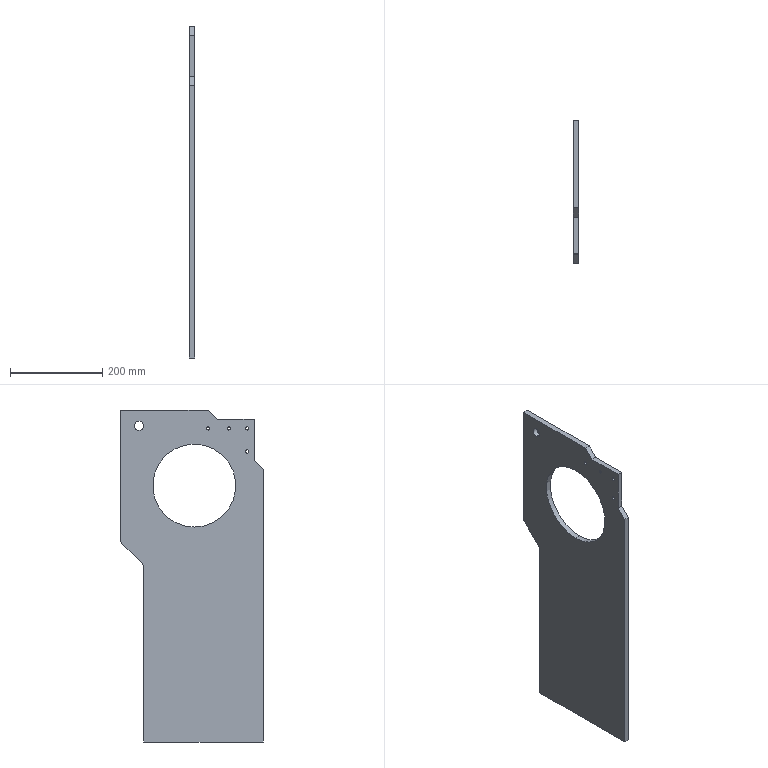Component | SolidWorks | JHK-A1003DriveWheelSupportPlateRight-3 | 1 solid | 28 faces | box 12 x 310 x 720 mm | volume 2071677 mm3 | cylinder 14 | plane 12 | cone 2 | commonest cylinder face diameters 6.8 x8 20 x4 180 x2 | material Q235A
build123d program:
from build123d import *

# Parameters (mm, degrees)
BOSS_EXTRUDE1_DEPTH = 6
SKETCH2_R           = 90
SKETCH2_R_2         = 10
CUT_EXTRUDE1_DEPTH  = 397.729
M8_TAPPED_HOLE1_D   = 6.8
FILLET1_R           = 10
CHAMFER1_SIZE       = 1.2


with BuildPart() as part:
    # Sketch1 → Boss-Extrude1 (new, symmetric)
    with BuildSketch(Plane(origin=(0, 0, 0), x_dir=(0, 0, -1), z_dir=(1, 0, 0))):
        Polygon((-355, 155), (-69, 155), (-19, 105), (365, 105), (365, -155), (-225, -155), (-245, -135), (-335, -135), (-335, -55), (-355, -35), align=None)
    extrude(amount=BOSS_EXTRUDE1_DEPTH, both=True)

    # Sketch2 → Cut-Extrude1 (cut, through all)
    with BuildSketch(Plane(origin=(6, 0, 0), x_dir=(0, 0, -1), z_dir=(1, 0, 0))):
        with Locations((-191, -5)):
            Circle(SKETCH2_R)
        with Locations((-321, 115)):
            Circle(SKETCH2_R_2)
    extrude(amount=-CUT_EXTRUDE1_DEPTH, mode=Mode.SUBTRACT)

    # M8 Tapped Hole1 (through all)
    with Locations(Plane(origin=(6, 0, 0), x_dir=(0, 0, -1), z_dir=(1, 0, 0))):
        with Locations((-315, -120), (-265, -120), (-315, -80), (-315, -35)):
            Hole(M8_TAPPED_HOLE1_D / 2)

    # Fillet1
    fillet1_edges = [part.edges().sort_by_distance(p)[0] for p in [
        (0, 155, 69),
        (0, 105, 19),
    ]]
    fillet(fillet1_edges, radius=FILLET1_R)

    # Chamfer1
    chamfer1_edges = [part.edges().sort_by_distance(p)[0] for p in [
        (6, 115, 331),
    ]]
    chamfer(chamfer1_edges, length=CHAMFER1_SIZE)


solid = part.part

# Placed as in the assembly
solid = solid.moved(Location((79, 0, 0), (0, 0, 0)))
STEP:
#1=CARTESIAN_POINT('',(3.299,4.528,13.031));
#2=VERTEX_POINT('',#1);
#3=CARTESIAN_POINT('',(3.299,4.528,12.244));
#4=VERTEX_POINT('',#3);
#5=CARTESIAN_POINT('',(3.299,4.528,12.638));
#6=DIRECTION('',(1.,0.,0.));
#7=DIRECTION('',(0.,0.,1.));
#8=AXIS2_PLACEMENT_3D('',#5,#6,#7);
#9=CIRCLE('',#8,0.3937);
#10=EDGE_CURVE('',#2,#4,#9,.T.);
#11=ORIENTED_EDGE('',*,*,#10,.F.);
#12=CARTESIAN_POINT('',(3.346,4.528,13.079));
#13=VERTEX_POINT('',#12);
#14=CARTESIAN_POINT('',(3.299,4.528,13.031));
#15=DIRECTION('',(0.7071,0.,0.7071));
#16=VECTOR('',#15,39.37);
#17=LINE('',#14,#16);
#18=EDGE_CURVE('',#2,#13,#17,.T.);
#19=ORIENTED_EDGE('',*,*,#18,.T.);
#20=CARTESIAN_POINT('',(3.346,4.528,12.197));
#21=VERTEX_POINT('',#20);
#22=CARTESIAN_POINT('',(3.346,4.528,12.638));
#23=DIRECTION('',(-1.,0.,0.));
#24=DIRECTION('',(0.,0.,1.));
#25=AXIS2_PLACEMENT_3D('',#22,#23,#24);
#26=CIRCLE('',#25,0.4409);
#27=EDGE_CURVE('',#21,#13,#26,.T.);
#28=ORIENTED_EDGE('',*,*,#27,.F.);
#29=CARTESIAN_POINT('',(3.299,4.528,12.244));
#30=DIRECTION('',(0.7071,0.,-0.7071));
#31=VECTOR('',#30,39.37);
#32=LINE('',#29,#31);
#33=EDGE_CURVE('',#4,#21,#32,.T.);
#34=ORIENTED_EDGE('',*,*,#33,.F.);
#35=EDGE_LOOP('',(#11,#19,#28,#34));
#36=FACE_OUTER_BOUND('',#35,.T.);
#37=CARTESIAN_POINT('',(3.299,4.528,12.638));
#38=DIRECTION('',(1.,0.,0.));
#39=DIRECTION('',(0.,0.,-1.));
#40=AXIS2_PLACEMENT_3D('',#37,#38,#39);
#41=CONICAL_SURFACE('',#40,0.3937,0.7854);
#42=ADVANCED_FACE('',(#36),#41,.F.);
#43=CARTESIAN_POINT('',(2.874,-4.724,12.535));
#44=VERTEX_POINT('',#43);
#45=CARTESIAN_POINT('',(2.874,-4.724,12.268));
#46=VERTEX_POINT('',#45);
#47=CARTESIAN_POINT('',(2.874,-4.724,12.402));
#48=DIRECTION('',(1.,0.,0.));
#49=DIRECTION('',(0.,0.,-1.));
#50=AXIS2_PLACEMENT_3D('',#47,#48,#49);
#51=CIRCLE('',#50,0.1339);
#52=EDGE_CURVE('',#44,#46,#51,.T.);
#53=ORIENTED_EDGE('',*,*,#52,.F.);
#54=CARTESIAN_POINT('',(3.346,-4.724,12.535));
#55=VERTEX_POINT('',#54);
#56=CARTESIAN_POINT('',(3.346,-4.724,12.535));
#57=DIRECTION('',(1.,0.,0.));
#58=VECTOR('',#57,39.37);
#59=LINE('',#56,#58);
#60=EDGE_CURVE('',#44,#55,#59,.T.);
#61=ORIENTED_EDGE('',*,*,#60,.T.);
#62=CARTESIAN_POINT('',(3.346,-4.724,12.268));
#63=VERTEX_POINT('',#62);
#64=CARTESIAN_POINT('',(3.346,-4.724,12.402));
#65=DIRECTION('',(1.,0.,0.));
#66=DIRECTION('',(0.,0.,-1.));
#67=AXIS2_PLACEMENT_3D('',#64,#65,#66);
#68=CIRCLE('',#67,0.1339);
#69=EDGE_CURVE('',#55,#63,#68,.T.);
#70=ORIENTED_EDGE('',*,*,#69,.T.);
#71=CARTESIAN_POINT('',(3.346,-4.724,12.268));
#72=DIRECTION('',(1.,0.,0.));
#73=VECTOR('',#72,39.37);
#74=LINE('',#71,#73);
#75=EDGE_CURVE('',#46,#63,#74,.T.);
#76=ORIENTED_EDGE('',*,*,#75,.F.);
#77=EDGE_LOOP('',(#53,#61,#70,#76));
#78=FACE_OUTER_BOUND('',#77,.T.);
#79=CARTESIAN_POINT('',(3.346,-4.724,12.402));
#80=DIRECTION('',(1.,0.,0.));
#81=DIRECTION('',(0.,0.,-1.));
#82=AXIS2_PLACEMENT_3D('',#79,#80,#81);
#83=CYLINDRICAL_SURFACE('',#82,0.1339);
#84=ADVANCED_FACE('',(#78),#83,.F.);
#85=CARTESIAN_POINT('',(2.874,-4.724,10.567));
#86=VERTEX_POINT('',#85);
#87=CARTESIAN_POINT('',(2.874,-4.724,10.299));
#88=VERTEX_POINT('',#87);
#89=CARTESIAN_POINT('',(2.874,-4.724,10.433));
#90=DIRECTION('',(1.,0.,0.));
#91=DIRECTION('',(0.,0.,-1.));
#92=AXIS2_PLACEMENT_3D('',#89,#90,#91);
#93=CIRCLE('',#92,0.1339);
#94=EDGE_CURVE('',#86,#88,#93,.T.);
#95=ORIENTED_EDGE('',*,*,#94,.F.);
#96=CARTESIAN_POINT('',(3.346,-4.724,10.567));
#97=VERTEX_POINT('',#96);
#98=CARTESIAN_POINT('',(3.346,-4.724,10.567));
#99=DIRECTION('',(1.,0.,0.));
#100=VECTOR('',#99,39.37);
#101=LINE('',#98,#100);
#102=EDGE_CURVE('',#86,#97,#101,.T.);
#103=ORIENTED_EDGE('',*,*,#102,.T.);
#104=CARTESIAN_POINT('',(3.346,-4.724,10.299));
#105=VERTEX_POINT('',#104);
#106=CARTESIAN_POINT('',(3.346,-4.724,10.433));
#107=DIRECTION('',(1.,0.,0.));
#108=DIRECTION('',(0.,0.,-1.));
#109=AXIS2_PLACEMENT_3D('',#106,#107,#108);
#110=CIRCLE('',#109,0.1339);
#111=EDGE_CURVE('',#97,#105,#110,.T.);
#112=ORIENTED_EDGE('',*,*,#111,.T.);
#113=CARTESIAN_POINT('',(3.346,-4.724,10.299));
#114=DIRECTION('',(1.,0.,0.));
#115=VECTOR('',#114,39.37);
#116=LINE('',#113,#115);
#117=EDGE_CURVE('',#88,#105,#116,.T.);
#118=ORIENTED_EDGE('',*,*,#117,.F.);
#119=EDGE_LOOP('',(#95,#103,#112,#118));
#120=FACE_OUTER_BOUND('',#119,.T.);
#121=CARTESIAN_POINT('',(3.346,-4.724,10.433));
#122=DIRECTION('',(1.,0.,0.));
#123=DIRECTION('',(0.,0.,-1.));
#124=AXIS2_PLACEMENT_3D('',#121,#122,#123);
#125=CYLINDRICAL_SURFACE('',#124,0.1339);
#126=ADVANCED_FACE('',(#120),#125,.F.);
#127=CARTESIAN_POINT('',(2.874,-3.15,12.535));
#128=VERTEX_POINT('',#127);
#129=CARTESIAN_POINT('',(2.874,-3.15,12.268));
#130=VERTEX_POINT('',#129);
#131=CARTESIAN_POINT('',(2.874,-3.15,12.402));
#132=DIRECTION('',(1.,0.,0.));
#133=DIRECTION('',(0.,0.,-1.));
#134=AXIS2_PLACEMENT_3D('',#131,#132,#133);
#135=CIRCLE('',#134,0.1339);
#136=EDGE_CURVE('',#128,#130,#135,.T.);
#137=ORIENTED_EDGE('',*,*,#136,.F.);
#138=CARTESIAN_POINT('',(3.346,-3.15,12.535));
#139=VERTEX_POINT('',#138);
#140=CARTESIAN_POINT('',(3.346,-3.15,12.535));
#141=DIRECTION('',(1.,0.,0.));
#142=VECTOR('',#141,39.37);
#143=LINE('',#140,#142);
#144=EDGE_CURVE('',#128,#139,#143,.T.);
#145=ORIENTED_EDGE('',*,*,#144,.T.);
#146=CARTESIAN_POINT('',(3.346,-3.15,12.268));
#147=VERTEX_POINT('',#146);
#148=CARTESIAN_POINT('',(3.346,-3.15,12.402));
#149=DIRECTION('',(1.,0.,0.));
#150=DIRECTION('',(0.,0.,-1.));
#151=AXIS2_PLACEMENT_3D('',#148,#149,#150);
#152=CIRCLE('',#151,0.1339);
#153=EDGE_CURVE('',#139,#147,#152,.T.);
#154=ORIENTED_EDGE('',*,*,#153,.T.);
#155=CARTESIAN_POINT('',(3.346,-3.15,12.268));
#156=DIRECTION('',(1.,0.,0.));
#157=VECTOR('',#156,39.37);
#158=LINE('',#155,#157);
#159=EDGE_CURVE('',#130,#147,#158,.T.);
#160=ORIENTED_EDGE('',*,*,#159,.F.);
#161=EDGE_LOOP('',(#137,#145,#154,#160));
#162=FACE_OUTER_BOUND('',#161,.T.);
#163=CARTESIAN_POINT('',(3.346,-3.15,12.402));
#164=DIRECTION('',(1.,0.,0.));
#165=DIRECTION('',(0.,0.,-1.));
#166=AXIS2_PLACEMENT_3D('',#163,#164,#165);
#167=CYLINDRICAL_SURFACE('',#166,0.1339);
#168=ADVANCED_FACE('',(#162),#167,.F.);
#169=CARTESIAN_POINT('',(2.874,-1.378,12.535));
#170=VERTEX_POINT('',#169);
#171=CARTESIAN_POINT('',(2.874,-1.378,12.268));
#172=VERTEX_POINT('',#171);
#173=CARTESIAN_POINT('',(2.874,-1.378,12.402));
#174=DIRECTION('',(1.,0.,0.));
#175=DIRECTION('',(0.,0.,-1.));
#176=AXIS2_PLACEMENT_3D('',#173,#174,#175);
#177=CIRCLE('',#176,0.1339);
#178=EDGE_CURVE('',#170,#172,#177,.T.);
#179=ORIENTED_EDGE('',*,*,#178,.F.);
#180=CARTESIAN_POINT('',(3.346,-1.378,12.535));
#181=VERTEX_POINT('',#180);
#182=CARTESIAN_POINT('',(3.346,-1.378,12.535));
#183=DIRECTION('',(1.,0.,0.));
#184=VECTOR('',#183,39.37);
#185=LINE('',#182,#184);
#186=EDGE_CURVE('',#170,#181,#185,.T.);
#187=ORIENTED_EDGE('',*,*,#186,.T.);
#188=CARTESIAN_POINT('',(3.346,-1.378,12.268));
#189=VERTEX_POINT('',#188);
#190=CARTESIAN_POINT('',(3.346,-1.378,12.402));
#191=DIRECTION('',(1.,0.,0.));
#192=DIRECTION('',(0.,0.,-1.));
#193=AXIS2_PLACEMENT_3D('',#190,#191,#192);
#194=CIRCLE('',#193,0.1339);
#195=EDGE_CURVE('',#181,#189,#194,.T.);
#196=ORIENTED_EDGE('',*,*,#195,.T.);
#197=CARTESIAN_POINT('',(3.346,-1.378,12.268));
#198=DIRECTION('',(1.,0.,0.));
#199=VECTOR('',#198,39.37);
#200=LINE('',#197,#199);
#201=EDGE_CURVE('',#172,#189,#200,.T.);
#202=ORIENTED_EDGE('',*,*,#201,.F.);
#203=EDGE_LOOP('',(#179,#187,#196,#202));
#204=FACE_OUTER_BOUND('',#203,.T.);
#205=CARTESIAN_POINT('',(3.346,-1.378,12.402));
#206=DIRECTION('',(1.,0.,0.));
#207=DIRECTION('',(0.,0.,-1.));
#208=AXIS2_PLACEMENT_3D('',#205,#206,#207);
#209=CYLINDRICAL_SURFACE('',#208,0.1339);
#210=ADVANCED_FACE('',(#204),#209,.F.);
#211=CARTESIAN_POINT('',(2.874,4.528,13.031));
#212=VERTEX_POINT('',#211);
#213=CARTESIAN_POINT('',(2.874,4.528,12.244));
#214=VERTEX_POINT('',#213);
#215=CARTESIAN_POINT('',(2.874,4.528,12.638));
#216=DIRECTION('',(1.,0.,0.));
#217=DIRECTION('',(0.,0.,-1.));
#218=AXIS2_PLACEMENT_3D('',#215,#216,#217);
#219=CIRCLE('',#218,0.3937);
#220=EDGE_CURVE('',#212,#214,#219,.T.);
#221=ORIENTED_EDGE('',*,*,#220,.F.);
#222=CARTESIAN_POINT('',(2.874,4.528,13.031));
#223=DIRECTION('',(1.,0.,0.));
#224=VECTOR('',#223,39.37);
#225=LINE('',#222,#224);
#226=EDGE_CURVE('',#212,#2,#225,.T.);
#227=ORIENTED_EDGE('',*,*,#226,.T.);
#228=ORIENTED_EDGE('',*,*,#10,.T.);
#229=CARTESIAN_POINT('',(2.874,4.528,12.244));
#230=DIRECTION('',(1.,0.,0.));
#231=VECTOR('',#230,39.37);
#232=LINE('',#229,#231);
#233=EDGE_CURVE('',#214,#4,#232,.T.);
#234=ORIENTED_EDGE('',*,*,#233,.F.);
#235=EDGE_LOOP('',(#221,#227,#228,#234));
#236=FACE_OUTER_BOUND('',#235,.T.);
#237=CARTESIAN_POINT('',(2.874,4.528,12.638));
#238=DIRECTION('',(1.,0.,0.));
#239=DIRECTION('',(0.,0.,-1.));
#240=AXIS2_PLACEMENT_3D('',#237,#238,#239);
#241=CYLINDRICAL_SURFACE('',#240,0.3937);
#242=ADVANCED_FACE('',(#236),#241,.F.);
#243=CARTESIAN_POINT('',(2.874,-0.1969,11.063));
#244=VERTEX_POINT('',#243);
#245=CARTESIAN_POINT('',(2.874,-0.1969,3.976));
#246=VERTEX_POINT('',#245);
#247=CARTESIAN_POINT('',(2.874,-0.1969,7.52));
#248=DIRECTION('',(1.,0.,0.));
#249=DIRECTION('',(0.,0.,-1.));
#250=AXIS2_PLACEMENT_3D('',#247,#248,#249);
#251=CIRCLE('',#250,3.543);
#252=EDGE_CURVE('',#244,#246,#251,.T.);
#253=ORIENTED_EDGE('',*,*,#252,.F.);
#254=CARTESIAN_POINT('',(3.346,-0.1969,11.063));
#255=VERTEX_POINT('',#254);
#256=CARTESIAN_POINT('',(2.874,-0.1969,11.063));
#257=DIRECTION('',(1.,0.,0.));
#258=VECTOR('',#257,39.37);
#259=LINE('',#256,#258);
#260=EDGE_CURVE('',#244,#255,#259,.T.);
#261=ORIENTED_EDGE('',*,*,#260,.T.);
#262=CARTESIAN_POINT('',(3.346,-0.1969,3.976));
#263=VERTEX_POINT('',#262);
#264=CARTESIAN_POINT('',(3.346,-0.1969,7.52));
#265=DIRECTION('',(1.,0.,0.));
#266=DIRECTION('',(0.,0.,-1.));
#267=AXIS2_PLACEMENT_3D('',#264,#265,#266);
#268=CIRCLE('',#267,3.543);
#269=EDGE_CURVE('',#255,#263,#268,.T.);
#270=ORIENTED_EDGE('',*,*,#269,.T.);
#271=CARTESIAN_POINT('',(2.874,-0.1969,3.976));
#272=DIRECTION('',(1.,0.,0.));
#273=VECTOR('',#272,39.37);
#274=LINE('',#271,#273);
#275=EDGE_CURVE('',#246,#263,#274,.T.);
#276=ORIENTED_EDGE('',*,*,#275,.F.);
#277=EDGE_LOOP('',(#253,#261,#270,#276));
#278=FACE_OUTER_BOUND('',#277,.T.);
#279=CARTESIAN_POINT('',(2.874,-0.1969,7.52));
#280=DIRECTION('',(1.,0.,0.));
#281=DIRECTION('',(0.,0.,-1.));
#282=AXIS2_PLACEMENT_3D('',#279,#280,#281);
#283=CYLINDRICAL_SURFACE('',#282,3.543);
#284=ADVANCED_FACE('',(#278),#283,.F.);
#285=CARTESIAN_POINT('',(2.874,6.102,13.976));
#286=VERTEX_POINT('',#285);
#287=CARTESIAN_POINT('',(2.874,-1.378,13.976));
#288=VERTEX_POINT('',#287);
#289=CARTESIAN_POINT('',(2.874,-1.378,13.976));
#290=DIRECTION('',(0.,-1.,0.));
#291=VECTOR('',#290,39.37);
#292=LINE('',#289,#291);
#293=EDGE_CURVE('',#286,#288,#292,.T.);
#294=ORIENTED_EDGE('',*,*,#293,.T.);
#295=CARTESIAN_POINT('',(3.346,-1.378,13.976));
#296=VERTEX_POINT('',#295);
#297=CARTESIAN_POINT('',(3.346,-1.378,13.976));
#298=DIRECTION('',(-1.,0.,0.));
#299=VECTOR('',#298,39.37);
#300=LINE('',#297,#299);
#301=EDGE_CURVE('',#296,#288,#300,.T.);
#302=ORIENTED_EDGE('',*,*,#301,.F.);
#303=CARTESIAN_POINT('',(3.346,6.102,13.976));
#304=VERTEX_POINT('',#303);
#305=CARTESIAN_POINT('',(3.346,-1.378,13.976));
#306=DIRECTION('',(0.,-1.,0.));
#307=VECTOR('',#306,39.37);
#308=LINE('',#305,#307);
#309=EDGE_CURVE('',#304,#296,#308,.T.);
#310=ORIENTED_EDGE('',*,*,#309,.F.);
#311=CARTESIAN_POINT('',(3.346,6.102,13.976));
#312=DIRECTION('',(-1.,0.,0.));
#313=VECTOR('',#312,39.37);
#314=LINE('',#311,#313);
#315=EDGE_CURVE('',#304,#286,#314,.T.);
#316=ORIENTED_EDGE('',*,*,#315,.T.);
#317=EDGE_LOOP('',(#294,#302,#310,#316));
#318=FACE_OUTER_BOUND('',#317,.T.);
#319=CARTESIAN_POINT('',(3.346,-1.378,13.976));
#320=DIRECTION('',(0.,0.,-1.));
#321=DIRECTION('',(-1.,0.,0.));
#322=AXIS2_PLACEMENT_3D('',#319,#320,#321);
#323=PLANE('',#322);
#324=ADVANCED_FACE('',(#318),#323,.F.);
#325=CARTESIAN_POINT('',(2.874,-2.165,13.189));
#326=VERTEX_POINT('',#325);
#327=CARTESIAN_POINT('',(2.874,-2.165,13.189));
#328=DIRECTION('',(0.,-0.7071,-0.7071));
#329=VECTOR('',#328,39.37);
#330=LINE('',#327,#329);
#331=EDGE_CURVE('',#288,#326,#330,.T.);
#332=ORIENTED_EDGE('',*,*,#331,.T.);
#333=CARTESIAN_POINT('',(3.346,-2.165,13.189));
#334=VERTEX_POINT('',#333);
#335=CARTESIAN_POINT('',(3.346,-2.165,13.189));
#336=DIRECTION('',(-1.,0.,0.));
#337=VECTOR('',#336,39.37);
#338=LINE('',#335,#337);
#339=EDGE_CURVE('',#334,#326,#338,.T.);
#340=ORIENTED_EDGE('',*,*,#339,.F.);
#341=CARTESIAN_POINT('',(3.346,-2.165,13.189));
#342=DIRECTION('',(0.,-0.7071,-0.7071));
#343=VECTOR('',#342,39.37);
#344=LINE('',#341,#343);
#345=EDGE_CURVE('',#296,#334,#344,.T.);
#346=ORIENTED_EDGE('',*,*,#345,.F.);
#347=ORIENTED_EDGE('',*,*,#301,.T.);
#348=EDGE_LOOP('',(#332,#340,#346,#347));
#349=FACE_OUTER_BOUND('',#348,.T.);
#350=CARTESIAN_POINT('',(3.346,-2.165,13.189));
#351=DIRECTION('',(0.,0.7071,-0.7071));
#352=DIRECTION('',(0.,0.7071,0.7071));
#353=AXIS2_PLACEMENT_3D('',#350,#351,#352);
#354=PLANE('',#353);
#355=ADVANCED_FACE('',(#349),#354,.F.);
#356=CARTESIAN_POINT('',(2.874,-5.315,13.189));
#357=VERTEX_POINT('',#356);
#358=CARTESIAN_POINT('',(2.874,-5.315,13.189));
#359=DIRECTION('',(0.,-1.,-0.));
#360=VECTOR('',#359,39.37);
#361=LINE('',#358,#360);
#362=EDGE_CURVE('',#326,#357,#361,.T.);
#363=ORIENTED_EDGE('',*,*,#362,.T.);
#364=CARTESIAN_POINT('',(3.346,-5.315,13.189));
#365=VERTEX_POINT('',#364);
#366=CARTESIAN_POINT('',(3.346,-5.315,13.189));
#367=DIRECTION('',(-1.,0.,0.));
#368=VECTOR('',#367,39.37);
#369=LINE('',#366,#368);
#370=EDGE_CURVE('',#365,#357,#369,.T.);
#371=ORIENTED_EDGE('',*,*,#370,.F.);
#372=CARTESIAN_POINT('',(3.346,-5.315,13.189));
#373=DIRECTION('',(0.,-1.,-0.));
#374=VECTOR('',#373,39.37);
#375=LINE('',#372,#374);
#376=EDGE_CURVE('',#334,#365,#375,.T.);
#377=ORIENTED_EDGE('',*,*,#376,.F.);
#378=ORIENTED_EDGE('',*,*,#339,.T.);
#379=EDGE_LOOP('',(#363,#371,#377,#378));
#380=FACE_OUTER_BOUND('',#379,.T.);
#381=CARTESIAN_POINT('',(3.346,-5.315,13.189));
#382=DIRECTION('',(0.,0.,-1.));
#383=DIRECTION('',(0.,1.,0.));
#384=AXIS2_PLACEMENT_3D('',#381,#382,#383);
#385=PLANE('',#384);
#386=ADVANCED_FACE('',(#380),#385,.F.);
#387=CARTESIAN_POINT('',(2.874,-5.315,9.646));
#388=VERTEX_POINT('',#387);
#389=CARTESIAN_POINT('',(2.874,-5.315,9.646));
#390=DIRECTION('',(0.,0.,-1.));
#391=VECTOR('',#390,39.37);
#392=LINE('',#389,#391);
#393=EDGE_CURVE('',#357,#388,#392,.T.);
#394=ORIENTED_EDGE('',*,*,#393,.T.);
#395=CARTESIAN_POINT('',(3.346,-5.315,9.646));
#396=VERTEX_POINT('',#395);
#397=CARTESIAN_POINT('',(3.346,-5.315,9.646));
#398=DIRECTION('',(-1.,0.,0.));
#399=VECTOR('',#398,39.37);
#400=LINE('',#397,#399);
#401=EDGE_CURVE('',#396,#388,#400,.T.);
#402=ORIENTED_EDGE('',*,*,#401,.F.);
#403=CARTESIAN_POINT('',(3.346,-5.315,9.646));
#404=DIRECTION('',(0.,0.,-1.));
#405=VECTOR('',#404,39.37);
#406=LINE('',#403,#405);
#407=EDGE_CURVE('',#365,#396,#406,.T.);
#408=ORIENTED_EDGE('',*,*,#407,.F.);
#409=ORIENTED_EDGE('',*,*,#370,.T.);
#410=EDGE_LOOP('',(#394,#402,#408,#409));
#411=FACE_OUTER_BOUND('',#410,.T.);
#412=CARTESIAN_POINT('',(3.346,-5.315,9.646));
#413=DIRECTION('',(0.,1.,0.));
#414=DIRECTION('',(0.,0.,1.));
#415=AXIS2_PLACEMENT_3D('',#412,#413,#414);
#416=PLANE('',#415);
#417=ADVANCED_FACE('',(#411),#416,.F.);
#418=CARTESIAN_POINT('',(2.874,-6.102,8.858));
#419=VERTEX_POINT('',#418);
#420=CARTESIAN_POINT('',(2.874,-6.102,8.858));
#421=DIRECTION('',(0.,-0.7071,-0.7071));
#422=VECTOR('',#421,39.37);
#423=LINE('',#420,#422);
#424=EDGE_CURVE('',#388,#419,#423,.T.);
#425=ORIENTED_EDGE('',*,*,#424,.T.);
#426=CARTESIAN_POINT('',(3.346,-6.102,8.858));
#427=VERTEX_POINT('',#426);
#428=CARTESIAN_POINT('',(3.346,-6.102,8.858));
#429=DIRECTION('',(-1.,0.,0.));
#430=VECTOR('',#429,39.37);
#431=LINE('',#428,#430);
#432=EDGE_CURVE('',#427,#419,#431,.T.);
#433=ORIENTED_EDGE('',*,*,#432,.F.);
#434=CARTESIAN_POINT('',(3.346,-6.102,8.858));
#435=DIRECTION('',(0.,-0.7071,-0.7071));
#436=VECTOR('',#435,39.37);
#437=LINE('',#434,#436);
#438=EDGE_CURVE('',#396,#427,#437,.T.);
#439=ORIENTED_EDGE('',*,*,#438,.F.);
#440=ORIENTED_EDGE('',*,*,#401,.T.);
#441=EDGE_LOOP('',(#425,#433,#439,#440));
#442=FACE_OUTER_BOUND('',#441,.T.);
#443=CARTESIAN_POINT('',(3.346,-6.102,8.858));
#444=DIRECTION('',(0.,0.7071,-0.7071));
#445=DIRECTION('',(0.,0.7071,0.7071));
#446=AXIS2_PLACEMENT_3D('',#443,#444,#445);
#447=PLANE('',#446);
#448=ADVANCED_FACE('',(#442),#447,.F.);
#449=CARTESIAN_POINT('',(2.874,-6.102,-14.37));
#450=VERTEX_POINT('',#449);
#451=CARTESIAN_POINT('',(2.874,-6.102,-14.37));
#452=DIRECTION('',(0.,0.,-1.));
#453=VECTOR('',#452,39.37);
#454=LINE('',#451,#453);
#455=EDGE_CURVE('',#419,#450,#454,.T.);
#456=ORIENTED_EDGE('',*,*,#455,.T.);
#457=CARTESIAN_POINT('',(3.346,-6.102,-14.37));
#458=VERTEX_POINT('',#457);
#459=CARTESIAN_POINT('',(3.346,-6.102,-14.37));
#460=DIRECTION('',(-1.,0.,0.));
#461=VECTOR('',#460,39.37);
#462=LINE('',#459,#461);
#463=EDGE_CURVE('',#458,#450,#462,.T.);
#464=ORIENTED_EDGE('',*,*,#463,.F.);
#465=CARTESIAN_POINT('',(3.346,-6.102,-14.37));
#466=DIRECTION('',(0.,0.,-1.));
#467=VECTOR('',#466,39.37);
#468=LINE('',#465,#467);
#469=EDGE_CURVE('',#427,#458,#468,.T.);
#470=ORIENTED_EDGE('',*,*,#469,.F.);
#471=ORIENTED_EDGE('',*,*,#432,.T.);
#472=EDGE_LOOP('',(#456,#464,#470,#471));
#473=FACE_OUTER_BOUND('',#472,.T.);
#474=CARTESIAN_POINT('',(3.346,-6.102,-14.37));
#475=DIRECTION('',(0.,1.,0.));
#476=DIRECTION('',(0.,-0.,1.));
#477=AXIS2_PLACEMENT_3D('',#474,#475,#476);
#478=PLANE('',#477);
#479=ADVANCED_FACE('',(#473),#478,.F.);
#480=CARTESIAN_POINT('',(2.874,4.134,-14.37));
#481=VERTEX_POINT('',#480);
#482=CARTESIAN_POINT('',(2.874,4.134,-14.37));
#483=DIRECTION('',(0.,1.,0.));
#484=VECTOR('',#483,39.37);
#485=LINE('',#482,#484);
#486=EDGE_CURVE('',#450,#481,#485,.T.);
#487=ORIENTED_EDGE('',*,*,#486,.T.);
#488=CARTESIAN_POINT('',(3.346,4.134,-14.37));
#489=VERTEX_POINT('',#488);
#490=CARTESIAN_POINT('',(3.346,4.134,-14.37));
#491=DIRECTION('',(-1.,0.,0.));
#492=VECTOR('',#491,39.37);
#493=LINE('',#490,#492);
#494=EDGE_CURVE('',#489,#481,#493,.T.);
#495=ORIENTED_EDGE('',*,*,#494,.F.);
#496=CARTESIAN_POINT('',(3.346,4.134,-14.37));
#497=DIRECTION('',(0.,1.,0.));
#498=VECTOR('',#497,39.37);
#499=LINE('',#496,#498);
#500=EDGE_CURVE('',#458,#489,#499,.T.);
#501=ORIENTED_EDGE('',*,*,#500,.F.);
#502=ORIENTED_EDGE('',*,*,#463,.T.);
#503=EDGE_LOOP('',(#487,#495,#501,#502));
#504=FACE_OUTER_BOUND('',#503,.T.);
#505=CARTESIAN_POINT('',(3.346,4.134,-14.37));
#506=DIRECTION('',(0.,-0.,1.));
#507=DIRECTION('',(0.,-1.,-0.));
#508=AXIS2_PLACEMENT_3D('',#505,#506,#507);
#509=PLANE('',#508);
#510=ADVANCED_FACE('',(#504),#509,.F.);
#511=CARTESIAN_POINT('',(2.874,4.134,0.585));
#512=VERTEX_POINT('',#511);
#513=CARTESIAN_POINT('',(2.874,4.134,0.748));
#514=DIRECTION('',(0.,0.,1.));
#515=VECTOR('',#514,39.37);
#516=LINE('',#513,#515);
#517=EDGE_CURVE('',#481,#512,#516,.T.);
#518=ORIENTED_EDGE('',*,*,#517,.T.);
#519=CARTESIAN_POINT('',(3.346,4.134,0.585));
#520=VERTEX_POINT('',#519);
#521=CARTESIAN_POINT('',(3.346,4.134,0.585));
#522=DIRECTION('',(1.,0.,0.));
#523=VECTOR('',#522,39.37);
#524=LINE('',#521,#523);
#525=EDGE_CURVE('',#512,#520,#524,.T.);
#526=ORIENTED_EDGE('',*,*,#525,.T.);
#527=CARTESIAN_POINT('',(3.346,4.134,0.748));
#528=DIRECTION('',(0.,0.,1.));
#529=VECTOR('',#528,39.37);
#530=LINE('',#527,#529);
#531=EDGE_CURVE('',#489,#520,#530,.T.);
#532=ORIENTED_EDGE('',*,*,#531,.F.);
#533=ORIENTED_EDGE('',*,*,#494,.T.);
#534=EDGE_LOOP('',(#518,#526,#532,#533));
#535=FACE_OUTER_BOUND('',#534,.T.);
#536=CARTESIAN_POINT('',(3.346,4.134,0.748));
#537=DIRECTION('',(0.,-1.,0.));
#538=DIRECTION('',(0.,0.,-1.));
#539=AXIS2_PLACEMENT_3D('',#536,#537,#538);
#540=PLANE('',#539);
#541=ADVANCED_FACE('',(#535),#540,.F.);
#542=CARTESIAN_POINT('',(2.874,4.249,0.8633));
#543=VERTEX_POINT('',#542);
#544=CARTESIAN_POINT('',(2.874,5.987,2.601));
#545=VERTEX_POINT('',#544);
#546=CARTESIAN_POINT('',(2.874,6.102,2.717));
#547=DIRECTION('',(0.,0.7071,0.7071));
#548=VECTOR('',#547,39.37);
#549=LINE('',#546,#548);
#550=EDGE_CURVE('',#543,#545,#549,.T.);
#551=ORIENTED_EDGE('',*,*,#550,.T.);
#552=CARTESIAN_POINT('',(3.346,5.987,2.601));
#553=VERTEX_POINT('',#552);
#554=CARTESIAN_POINT('',(3.346,5.987,2.601));
#555=DIRECTION('',(1.,0.,0.));
#556=VECTOR('',#555,39.37);
#557=LINE('',#554,#556);
#558=EDGE_CURVE('',#545,#553,#557,.T.);
#559=ORIENTED_EDGE('',*,*,#558,.T.);
#560=CARTESIAN_POINT('',(3.346,4.249,0.8633));
#561=VERTEX_POINT('',#560);
#562=CARTESIAN_POINT('',(3.346,6.102,2.717));
#563=DIRECTION('',(0.,0.7071,0.7071));
#564=VECTOR('',#563,39.37);
#565=LINE('',#562,#564);
#566=EDGE_CURVE('',#561,#553,#565,.T.);
#567=ORIENTED_EDGE('',*,*,#566,.F.);
#568=CARTESIAN_POINT('',(2.874,4.249,0.8633));
#569=DIRECTION('',(-1.,0.,0.));
#570=VECTOR('',#569,39.37);
#571=LINE('',#568,#570);
#572=EDGE_CURVE('',#561,#543,#571,.T.);
#573=ORIENTED_EDGE('',*,*,#572,.T.);
#574=EDGE_LOOP('',(#551,#559,#567,#573));
#575=FACE_OUTER_BOUND('',#574,.T.);
#576=CARTESIAN_POINT('',(3.346,6.102,2.717));
#577=DIRECTION('',(0.,-0.7071,0.7071));
#578=DIRECTION('',(0.,-0.7071,-0.7071));
#579=AXIS2_PLACEMENT_3D('',#576,#577,#578);
#580=PLANE('',#579);
#581=ADVANCED_FACE('',(#575),#580,.F.);
#582=CARTESIAN_POINT('',(3.346,6.102,2.88));
#583=VERTEX_POINT('',#582);
#584=CARTESIAN_POINT('',(3.346,6.102,13.976));
#585=DIRECTION('',(0.,0.,1.));
#586=VECTOR('',#585,39.37);
#587=LINE('',#584,#586);
#588=EDGE_CURVE('',#583,#304,#587,.T.);
#589=ORIENTED_EDGE('',*,*,#588,.F.);
#590=CARTESIAN_POINT('',(2.874,6.102,2.88));
#591=VERTEX_POINT('',#590);
#592=CARTESIAN_POINT('',(3.346,6.102,2.88));
#593=DIRECTION('',(-1.,0.,0.));
#594=VECTOR('',#593,39.37);
#595=LINE('',#592,#594);
#596=EDGE_CURVE('',#583,#591,#595,.T.);
#597=ORIENTED_EDGE('',*,*,#596,.T.);
#598=CARTESIAN_POINT('',(2.874,6.102,13.976));
#599=DIRECTION('',(0.,0.,1.));
#600=VECTOR('',#599,39.37);
#601=LINE('',#598,#600);
#602=EDGE_CURVE('',#591,#286,#601,.T.);
#603=ORIENTED_EDGE('',*,*,#602,.T.);
#604=ORIENTED_EDGE('',*,*,#315,.F.);
#605=EDGE_LOOP('',(#589,#597,#603,#604));
#606=FACE_OUTER_BOUND('',#605,.T.);
#607=CARTESIAN_POINT('',(3.346,6.102,13.976));
#608=DIRECTION('',(0.,-1.,0.));
#609=DIRECTION('',(0.,0.,-1.));
#610=AXIS2_PLACEMENT_3D('',#607,#608,#609);
#611=PLANE('',#610);
#612=ADVANCED_FACE('',(#606),#611,.F.);
#613=ORIENTED_EDGE('',*,*,#27,.T.);
#614=CARTESIAN_POINT('',(3.346,4.528,12.638));
#615=DIRECTION('',(-1.,0.,0.));
#616=DIRECTION('',(0.,0.,1.));
#617=AXIS2_PLACEMENT_3D('',#614,#615,#616);
#618=CIRCLE('',#617,0.4409);
#619=EDGE_CURVE('',#13,#21,#618,.T.);
#620=ORIENTED_EDGE('',*,*,#619,.T.);
#621=EDGE_LOOP('',(#613,#620));
#622=FACE_BOUND('',#621,.T.);
#623=CARTESIAN_POINT('',(3.346,-4.724,12.402));
#624=DIRECTION('',(1.,0.,0.));
#625=DIRECTION('',(0.,0.,-1.));
#626=AXIS2_PLACEMENT_3D('',#623,#624,#625);
#627=CIRCLE('',#626,0.1339);
#628=EDGE_CURVE('',#63,#55,#627,.T.);
#629=ORIENTED_EDGE('',*,*,#628,.F.);
#630=ORIENTED_EDGE('',*,*,#69,.F.);
#631=EDGE_LOOP('',(#629,#630));
#632=FACE_BOUND('',#631,.T.);
#633=CARTESIAN_POINT('',(3.346,-4.724,10.433));
#634=DIRECTION('',(1.,0.,0.));
#635=DIRECTION('',(0.,0.,-1.));
#636=AXIS2_PLACEMENT_3D('',#633,#634,#635);
#637=CIRCLE('',#636,0.1339);
#638=EDGE_CURVE('',#105,#97,#637,.T.);
#639=ORIENTED_EDGE('',*,*,#638,.F.);
#640=ORIENTED_EDGE('',*,*,#111,.F.);
#641=EDGE_LOOP('',(#639,#640));
#642=FACE_BOUND('',#641,.T.);
#643=CARTESIAN_POINT('',(3.346,-3.15,12.402));
#644=DIRECTION('',(1.,0.,0.));
#645=DIRECTION('',(0.,0.,-1.));
#646=AXIS2_PLACEMENT_3D('',#643,#644,#645);
#647=CIRCLE('',#646,0.1339);
#648=EDGE_CURVE('',#147,#139,#647,.T.);
#649=ORIENTED_EDGE('',*,*,#648,.F.);
#650=ORIENTED_EDGE('',*,*,#153,.F.);
#651=EDGE_LOOP('',(#649,#650));
#652=FACE_BOUND('',#651,.T.);
#653=CARTESIAN_POINT('',(3.346,-1.378,12.402));
#654=DIRECTION('',(1.,0.,0.));
#655=DIRECTION('',(0.,0.,-1.));
#656=AXIS2_PLACEMENT_3D('',#653,#654,#655);
#657=CIRCLE('',#656,0.1339);
#658=EDGE_CURVE('',#189,#181,#657,.T.);
#659=ORIENTED_EDGE('',*,*,#658,.F.);
#660=ORIENTED_EDGE('',*,*,#195,.F.);
#661=EDGE_LOOP('',(#659,#660));
#662=FACE_BOUND('',#661,.T.);
#663=CARTESIAN_POINT('',(3.346,-0.1969,7.52));
#664=DIRECTION('',(1.,0.,0.));
#665=DIRECTION('',(0.,0.,-1.));
#666=AXIS2_PLACEMENT_3D('',#663,#664,#665);
#667=CIRCLE('',#666,3.543);
#668=EDGE_CURVE('',#263,#255,#667,.T.);
#669=ORIENTED_EDGE('',*,*,#668,.F.);
#670=ORIENTED_EDGE('',*,*,#269,.F.);
#671=EDGE_LOOP('',(#669,#670));
#672=FACE_BOUND('',#671,.T.);
#673=ORIENTED_EDGE('',*,*,#566,.T.);
#674=CARTESIAN_POINT('',(3.346,5.709,2.88));
#675=DIRECTION('',(1.,0.,0.));
#676=DIRECTION('',(0.,0.,1.));
#677=AXIS2_PLACEMENT_3D('',#674,#675,#676);
#678=CIRCLE('',#677,0.3937);
#679=EDGE_CURVE('',#553,#583,#678,.T.);
#680=ORIENTED_EDGE('',*,*,#679,.T.);
#681=ORIENTED_EDGE('',*,*,#588,.T.);
#682=ORIENTED_EDGE('',*,*,#309,.T.);
#683=ORIENTED_EDGE('',*,*,#345,.T.);
#684=ORIENTED_EDGE('',*,*,#376,.T.);
#685=ORIENTED_EDGE('',*,*,#407,.T.);
#686=ORIENTED_EDGE('',*,*,#438,.T.);
#687=ORIENTED_EDGE('',*,*,#469,.T.);
#688=ORIENTED_EDGE('',*,*,#500,.T.);
#689=ORIENTED_EDGE('',*,*,#531,.T.);
#690=CARTESIAN_POINT('',(3.346,4.528,0.585));
#691=DIRECTION('',(-1.,0.,0.));
#692=DIRECTION('',(0.,0.,1.));
#693=AXIS2_PLACEMENT_3D('',#690,#691,#692);
#694=CIRCLE('',#693,0.3937);
#695=EDGE_CURVE('',#520,#561,#694,.T.);
#696=ORIENTED_EDGE('',*,*,#695,.T.);
#697=EDGE_LOOP('',(#673,#680,#681,#682,#683,#684,#685,#686,#687,#688,#689,#696));
#698=FACE_OUTER_BOUND('',#697,.T.);
#699=CARTESIAN_POINT('',(3.346,0.,0.));
#700=DIRECTION('',(-1.,0.,0.));
#701=DIRECTION('',(0.,0.,1.));
#702=AXIS2_PLACEMENT_3D('',#699,#700,#701);
#703=PLANE('',#702);
#704=ADVANCED_FACE('',(#622,#632,#642,#652,#662,#672,#698),#703,.F.);
#705=CARTESIAN_POINT('',(2.874,-4.724,12.402));
#706=DIRECTION('',(1.,0.,0.));
#707=DIRECTION('',(0.,0.,-1.));
#708=AXIS2_PLACEMENT_3D('',#705,#706,#707);
#709=CIRCLE('',#708,0.1339);
#710=EDGE_CURVE('',#46,#44,#709,.T.);
#711=ORIENTED_EDGE('',*,*,#710,.T.);
#712=ORIENTED_EDGE('',*,*,#52,.T.);
#713=EDGE_LOOP('',(#711,#712));
#714=FACE_BOUND('',#713,.T.);
#715=CARTESIAN_POINT('',(2.874,-4.724,10.433));
#716=DIRECTION('',(1.,0.,0.));
#717=DIRECTION('',(0.,0.,-1.));
#718=AXIS2_PLACEMENT_3D('',#715,#716,#717);
#719=CIRCLE('',#718,0.1339);
#720=EDGE_CURVE('',#88,#86,#719,.T.);
#721=ORIENTED_EDGE('',*,*,#720,.T.);
#722=ORIENTED_EDGE('',*,*,#94,.T.);
#723=EDGE_LOOP('',(#721,#722));
#724=FACE_BOUND('',#723,.T.);
#725=CARTESIAN_POINT('',(2.874,-3.15,12.402));
#726=DIRECTION('',(1.,0.,0.));
#727=DIRECTION('',(0.,0.,-1.));
#728=AXIS2_PLACEMENT_3D('',#725,#726,#727);
#729=CIRCLE('',#728,0.1339);
#730=EDGE_CURVE('',#130,#128,#729,.T.);
#731=ORIENTED_EDGE('',*,*,#730,.T.);
#732=ORIENTED_EDGE('',*,*,#136,.T.);
#733=EDGE_LOOP('',(#731,#732));
#734=FACE_BOUND('',#733,.T.);
#735=CARTESIAN_POINT('',(2.874,-1.378,12.402));
#736=DIRECTION('',(1.,0.,0.));
#737=DIRECTION('',(0.,0.,-1.));
#738=AXIS2_PLACEMENT_3D('',#735,#736,#737);
#739=CIRCLE('',#738,0.1339);
#740=EDGE_CURVE('',#172,#170,#739,.T.);
#741=ORIENTED_EDGE('',*,*,#740,.T.);
#742=ORIENTED_EDGE('',*,*,#178,.T.);
#743=EDGE_LOOP('',(#741,#742));
#744=FACE_BOUND('',#743,.T.);
#745=CARTESIAN_POINT('',(2.874,4.528,12.638));
#746=DIRECTION('',(1.,0.,0.));
#747=DIRECTION('',(0.,0.,-1.));
#748=AXIS2_PLACEMENT_3D('',#745,#746,#747);
#749=CIRCLE('',#748,0.3937);
#750=EDGE_CURVE('',#214,#212,#749,.T.);
#751=ORIENTED_EDGE('',*,*,#750,.T.);
#752=ORIENTED_EDGE('',*,*,#220,.T.);
#753=EDGE_LOOP('',(#751,#752));
#754=FACE_BOUND('',#753,.T.);
#755=CARTESIAN_POINT('',(2.874,-0.1969,7.52));
#756=DIRECTION('',(1.,0.,0.));
#757=DIRECTION('',(0.,0.,-1.));
#758=AXIS2_PLACEMENT_3D('',#755,#756,#757);
#759=CIRCLE('',#758,3.543);
#760=EDGE_CURVE('',#246,#244,#759,.T.);
#761=ORIENTED_EDGE('',*,*,#760,.T.);
#762=ORIENTED_EDGE('',*,*,#252,.T.);
#763=EDGE_LOOP('',(#761,#762));
#764=FACE_BOUND('',#763,.T.);
#765=ORIENTED_EDGE('',*,*,#602,.F.);
#766=CARTESIAN_POINT('',(2.874,5.709,2.88));
#767=DIRECTION('',(-1.,0.,0.));
#768=DIRECTION('',(0.,0.,1.));
#769=AXIS2_PLACEMENT_3D('',#766,#767,#768);
#770=CIRCLE('',#769,0.3937);
#771=EDGE_CURVE('',#591,#545,#770,.T.);
#772=ORIENTED_EDGE('',*,*,#771,.T.);
#773=ORIENTED_EDGE('',*,*,#550,.F.);
#774=CARTESIAN_POINT('',(2.874,4.528,0.585));
#775=DIRECTION('',(1.,0.,0.));
#776=DIRECTION('',(0.,0.,1.));
#777=AXIS2_PLACEMENT_3D('',#774,#775,#776);
#778=CIRCLE('',#777,0.3937);
#779=EDGE_CURVE('',#543,#512,#778,.T.);
#780=ORIENTED_EDGE('',*,*,#779,.T.);
#781=ORIENTED_EDGE('',*,*,#517,.F.);
#782=ORIENTED_EDGE('',*,*,#486,.F.);
#783=ORIENTED_EDGE('',*,*,#455,.F.);
#784=ORIENTED_EDGE('',*,*,#424,.F.);
#785=ORIENTED_EDGE('',*,*,#393,.F.);
#786=ORIENTED_EDGE('',*,*,#362,.F.);
#787=ORIENTED_EDGE('',*,*,#331,.F.);
#788=ORIENTED_EDGE('',*,*,#293,.F.);
#789=EDGE_LOOP('',(#765,#772,#773,#780,#781,#782,#783,#784,#785,#786,#787,#788));
#790=FACE_OUTER_BOUND('',#789,.T.);
#791=CARTESIAN_POINT('',(2.874,0.,0.));
#792=DIRECTION('',(-1.,0.,0.));
#793=DIRECTION('',(0.,0.,1.));
#794=AXIS2_PLACEMENT_3D('',#791,#792,#793);
#795=PLANE('',#794);
#796=ADVANCED_FACE('',(#714,#724,#734,#744,#754,#764,#790),#795,.T.);
#797=ORIENTED_EDGE('',*,*,#260,.F.);
#798=ORIENTED_EDGE('',*,*,#760,.F.);
#799=ORIENTED_EDGE('',*,*,#275,.T.);
#800=ORIENTED_EDGE('',*,*,#668,.T.);
#801=EDGE_LOOP('',(#797,#798,#799,#800));
#802=FACE_OUTER_BOUND('',#801,.T.);
#803=CARTESIAN_POINT('',(2.874,-0.1969,7.52));
#804=DIRECTION('',(1.,0.,0.));
#805=DIRECTION('',(0.,0.,-1.));
#806=AXIS2_PLACEMENT_3D('',#803,#804,#805);
#807=CYLINDRICAL_SURFACE('',#806,3.543);
#808=ADVANCED_FACE('',(#802),#807,.F.);
#809=ORIENTED_EDGE('',*,*,#226,.F.);
#810=ORIENTED_EDGE('',*,*,#750,.F.);
#811=ORIENTED_EDGE('',*,*,#233,.T.);
#812=CARTESIAN_POINT('',(3.299,4.528,12.638));
#813=DIRECTION('',(1.,0.,0.));
#814=DIRECTION('',(0.,0.,1.));
#815=AXIS2_PLACEMENT_3D('',#812,#813,#814);
#816=CIRCLE('',#815,0.3937);
#817=EDGE_CURVE('',#4,#2,#816,.T.);
#818=ORIENTED_EDGE('',*,*,#817,.T.);
#819=EDGE_LOOP('',(#809,#810,#811,#818));
#820=FACE_OUTER_BOUND('',#819,.T.);
#821=CARTESIAN_POINT('',(2.874,4.528,12.638));
#822=DIRECTION('',(1.,0.,0.));
#823=DIRECTION('',(0.,0.,-1.));
#824=AXIS2_PLACEMENT_3D('',#821,#822,#823);
#825=CYLINDRICAL_SURFACE('',#824,0.3937);
#826=ADVANCED_FACE('',(#820),#825,.F.);
#827=ORIENTED_EDGE('',*,*,#186,.F.);
#828=ORIENTED_EDGE('',*,*,#740,.F.);
#829=ORIENTED_EDGE('',*,*,#201,.T.);
#830=ORIENTED_EDGE('',*,*,#658,.T.);
#831=EDGE_LOOP('',(#827,#828,#829,#830));
#832=FACE_OUTER_BOUND('',#831,.T.);
#833=CARTESIAN_POINT('',(3.346,-1.378,12.402));
#834=DIRECTION('',(1.,0.,0.));
#835=DIRECTION('',(0.,0.,-1.));
#836=AXIS2_PLACEMENT_3D('',#833,#834,#835);
#837=CYLINDRICAL_SURFACE('',#836,0.1339);
#838=ADVANCED_FACE('',(#832),#837,.F.);
#839=ORIENTED_EDGE('',*,*,#144,.F.);
#840=ORIENTED_EDGE('',*,*,#730,.F.);
#841=ORIENTED_EDGE('',*,*,#159,.T.);
#842=ORIENTED_EDGE('',*,*,#648,.T.);
#843=EDGE_LOOP('',(#839,#840,#841,#842));
#844=FACE_OUTER_BOUND('',#843,.T.);
#845=CARTESIAN_POINT('',(3.346,-3.15,12.402));
#846=DIRECTION('',(1.,0.,0.));
#847=DIRECTION('',(0.,0.,-1.));
#848=AXIS2_PLACEMENT_3D('',#845,#846,#847);
#849=CYLINDRICAL_SURFACE('',#848,0.1339);
#850=ADVANCED_FACE('',(#844),#849,.F.);
#851=ORIENTED_EDGE('',*,*,#102,.F.);
#852=ORIENTED_EDGE('',*,*,#720,.F.);
#853=ORIENTED_EDGE('',*,*,#117,.T.);
#854=ORIENTED_EDGE('',*,*,#638,.T.);
#855=EDGE_LOOP('',(#851,#852,#853,#854));
#856=FACE_OUTER_BOUND('',#855,.T.);
#857=CARTESIAN_POINT('',(3.346,-4.724,10.433));
#858=DIRECTION('',(1.,0.,0.));
#859=DIRECTION('',(0.,0.,-1.));
#860=AXIS2_PLACEMENT_3D('',#857,#858,#859);
#861=CYLINDRICAL_SURFACE('',#860,0.1339);
#862=ADVANCED_FACE('',(#856),#861,.F.);
#863=ORIENTED_EDGE('',*,*,#60,.F.);
#864=ORIENTED_EDGE('',*,*,#710,.F.);
#865=ORIENTED_EDGE('',*,*,#75,.T.);
#866=ORIENTED_EDGE('',*,*,#628,.T.);
#867=EDGE_LOOP('',(#863,#864,#865,#866));
#868=FACE_OUTER_BOUND('',#867,.T.);
#869=CARTESIAN_POINT('',(3.346,-4.724,12.402));
#870=DIRECTION('',(1.,0.,0.));
#871=DIRECTION('',(0.,0.,-1.));
#872=AXIS2_PLACEMENT_3D('',#869,#870,#871);
#873=CYLINDRICAL_SURFACE('',#872,0.1339);
#874=ADVANCED_FACE('',(#868),#873,.F.);
#875=ORIENTED_EDGE('',*,*,#679,.F.);
#876=ORIENTED_EDGE('',*,*,#558,.F.);
#877=ORIENTED_EDGE('',*,*,#771,.F.);
#878=ORIENTED_EDGE('',*,*,#596,.F.);
#879=EDGE_LOOP('',(#875,#876,#877,#878));
#880=FACE_OUTER_BOUND('',#879,.T.);
#881=CARTESIAN_POINT('',(3.346,5.709,2.88));
#882=DIRECTION('',(-1.,0.,0.));
#883=DIRECTION('',(0.,0.,1.));
#884=AXIS2_PLACEMENT_3D('',#881,#882,#883);
#885=CYLINDRICAL_SURFACE('',#884,0.3937);
#886=ADVANCED_FACE('',(#880),#885,.T.);
#887=ORIENTED_EDGE('',*,*,#695,.F.);
#888=ORIENTED_EDGE('',*,*,#525,.F.);
#889=ORIENTED_EDGE('',*,*,#779,.F.);
#890=ORIENTED_EDGE('',*,*,#572,.F.);
#891=EDGE_LOOP('',(#887,#888,#889,#890));
#892=FACE_OUTER_BOUND('',#891,.T.);
#893=CARTESIAN_POINT('',(3.346,4.528,0.585));
#894=DIRECTION('',(1.,0.,0.));
#895=DIRECTION('',(0.,0.,-1.));
#896=AXIS2_PLACEMENT_3D('',#893,#894,#895);
#897=CYLINDRICAL_SURFACE('',#896,0.3937);
#898=ADVANCED_FACE('',(#892),#897,.F.);
#899=ORIENTED_EDGE('',*,*,#18,.F.);
#900=ORIENTED_EDGE('',*,*,#817,.F.);
#901=ORIENTED_EDGE('',*,*,#33,.T.);
#902=ORIENTED_EDGE('',*,*,#619,.F.);
#903=EDGE_LOOP('',(#899,#900,#901,#902));
#904=FACE_OUTER_BOUND('',#903,.T.);
#905=CARTESIAN_POINT('',(3.299,4.528,12.638));
#906=DIRECTION('',(1.,0.,0.));
#907=DIRECTION('',(0.,0.,-1.));
#908=AXIS2_PLACEMENT_3D('',#905,#906,#907);
#909=CONICAL_SURFACE('',#908,0.3937,0.7854);
#910=ADVANCED_FACE('',(#904),#909,.F.);
#911=CLOSED_SHELL('',(#42,#84,#126,#168,#210,#242,#284,#324,#355,#386,#417,#448,#479,#510,#541,#581,#612,#704,#796,#808,#826,#838,#850,#862,#874,#886,#898,#910));
#912=MANIFOLD_SOLID_BREP('',#911);
#913=CARTESIAN_POINT('',(0.,0.,0.));
#914=DIRECTION('',(0.,0.,1.));
#915=DIRECTION('',(1.,0.,0.));
#916=AXIS2_PLACEMENT_3D('',#913,#914,#915);
#917=(LENGTH_UNIT()NAMED_UNIT(*)SI_UNIT($,.METRE.));
#918=LENGTH_MEASURE_WITH_UNIT(LENGTH_MEASURE(0.0254),#917);
#919=DIMENSIONAL_EXPONENTS(1.,0.,0.,0.,0.,0.,0.);
#920=(CONVERSION_BASED_UNIT('',#918)LENGTH_UNIT()NAMED_UNIT(#919));
#921=UNCERTAINTY_MEASURE_WITH_UNIT(LENGTH_MEASURE(0.00001),#920,'','');
#922=(NAMED_UNIT(*)PLANE_ANGLE_UNIT()SI_UNIT($,.RADIAN.));
#923=(NAMED_UNIT(*)SI_UNIT($,.STERADIAN.)SOLID_ANGLE_UNIT());
#924=(GEOMETRIC_REPRESENTATION_CONTEXT(3)GLOBAL_UNCERTAINTY_ASSIGNED_CONTEXT((#921))GLOBAL_UNIT_ASSIGNED_CONTEXT((#920,#922,#923))REPRESENTATION_CONTEXT('',''));
#925=ADVANCED_BREP_SHAPE_REPRESENTATION('',(#912,#916),#924);
#926=COLOUR_RGB('',0.7922,0.8196,0.9333);
#927=FILL_AREA_STYLE_COLOUR('',#926);
#928=FILL_AREA_STYLE('',(#927));
#929=SURFACE_STYLE_FILL_AREA(#928);
#930=SURFACE_SIDE_STYLE('',(#929));
#931=SURFACE_STYLE_USAGE(.BOTH.,#930);
#932=PRESENTATION_STYLE_ASSIGNMENT((#931));
#933=STYLED_ITEM('',(#932),#912);
#934=(LENGTH_UNIT()NAMED_UNIT(*)SI_UNIT($,.METRE.));
#935=LENGTH_MEASURE_WITH_UNIT(LENGTH_MEASURE(0.0254),#934);
#936=DIMENSIONAL_EXPONENTS(1.,0.,0.,0.,0.,0.,0.);
#937=(CONVERSION_BASED_UNIT('',#935)LENGTH_UNIT()NAMED_UNIT(#936));
#938=UNCERTAINTY_MEASURE_WITH_UNIT(LENGTH_MEASURE(0.00001),#937,'','');
#939=(NAMED_UNIT(*)PLANE_ANGLE_UNIT()SI_UNIT($,.RADIAN.));
#940=(NAMED_UNIT(*)SI_UNIT($,.STERADIAN.)SOLID_ANGLE_UNIT());
#941=(GEOMETRIC_REPRESENTATION_CONTEXT(3)GLOBAL_UNCERTAINTY_ASSIGNED_CONTEXT((#938))GLOBAL_UNIT_ASSIGNED_CONTEXT((#937,#939,#940))REPRESENTATION_CONTEXT('',''));
#942=MECHANICAL_DESIGN_GEOMETRIC_PRESENTATION_REPRESENTATION('',(#933),#941);
#943=PRESENTATION_LAYER_ASSIGNMENT('','',(#933));